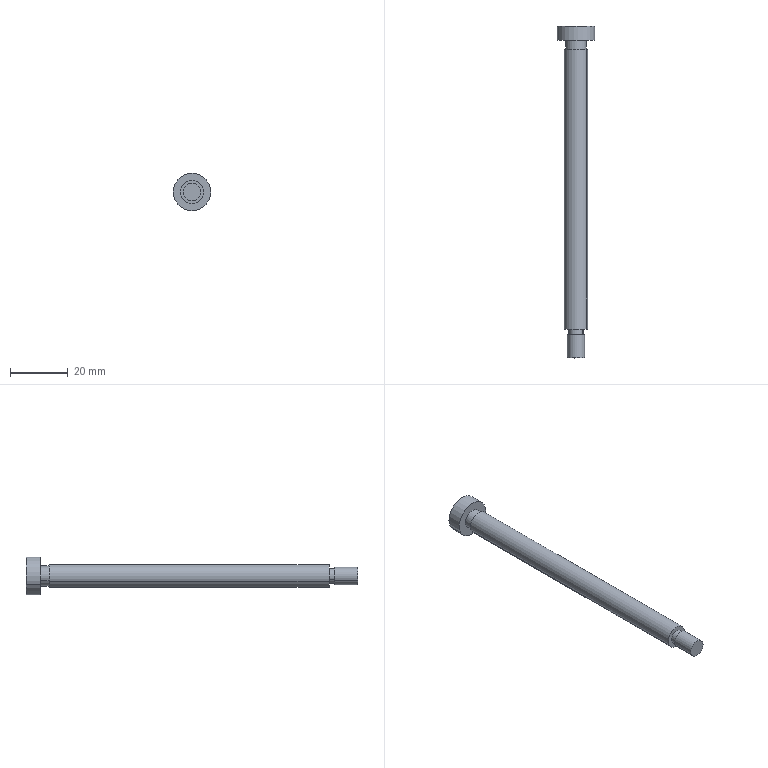Component | SolidWorks | ElectricalBoxAssembly2-1_M6-8-13-100GuidePinBolt-1 | 1 solid | 23 faces | box 13 x 115 x 13 mm | volume 5851 mm3 | plane 13 | cylinder 10 | commonest cylinder face diameters 6 x2 5 x2 13 x2 7 x2 8 x2
STEP:
#1=COLOUR_RGB('',0.7922,0.8196,0.9333);
#2=FILL_AREA_STYLE_COLOUR('',#1);
#3=FILL_AREA_STYLE('',(#2));
#4=SURFACE_STYLE_FILL_AREA(#3);
#5=SURFACE_SIDE_STYLE('',(#4));
#6=SURFACE_STYLE_USAGE(.BOTH.,#5);
#7=PRESENTATION_STYLE_ASSIGNMENT((#6));
#8=CARTESIAN_POINT('',(28.076,14.947,59.362));
#9=VERTEX_POINT('',#8);
#10=CARTESIAN_POINT('',(27.867,14.947,59.252));
#11=VERTEX_POINT('',#10);
#12=CARTESIAN_POINT('',(27.971,14.947,59.307));
#13=DIRECTION('',(0.,-1.,0.));
#14=DIRECTION('',(0.8849,0.,0.4657));
#15=AXIS2_PLACEMENT_3D('',#12,#13,#14);
#16=CIRCLE('',#15,0.1181);
#17=EDGE_CURVE('',#9,#11,#16,.T.);
#18=ORIENTED_EDGE('',*,*,#17,.F.);
#19=CARTESIAN_POINT('',(28.076,15.262,59.362));
#20=VERTEX_POINT('',#19);
#21=CARTESIAN_POINT('',(28.076,14.947,59.362));
#22=DIRECTION('',(-0.,1.,-0.));
#23=VECTOR('',#22,39.37);
#24=LINE('',#21,#23);
#25=EDGE_CURVE('',#9,#20,#24,.T.);
#26=ORIENTED_EDGE('',*,*,#25,.T.);
#27=CARTESIAN_POINT('',(27.867,15.262,59.252));
#28=VERTEX_POINT('',#27);
#29=CARTESIAN_POINT('',(27.971,15.262,59.307));
#30=DIRECTION('',(0.,-1.,0.));
#31=DIRECTION('',(0.8849,0.,0.4657));
#32=AXIS2_PLACEMENT_3D('',#29,#30,#31);
#33=CIRCLE('',#32,0.1181);
#34=EDGE_CURVE('',#20,#28,#33,.T.);
#35=ORIENTED_EDGE('',*,*,#34,.T.);
#36=CARTESIAN_POINT('',(27.867,14.947,59.252));
#37=DIRECTION('',(-0.,1.,-0.));
#38=VECTOR('',#37,39.37);
#39=LINE('',#36,#38);
#40=EDGE_CURVE('',#11,#28,#39,.T.);
#41=ORIENTED_EDGE('',*,*,#40,.F.);
#42=EDGE_LOOP('',(#18,#26,#35,#41));
#43=FACE_OUTER_BOUND('',#42,.T.);
#44=CARTESIAN_POINT('',(27.971,14.947,59.307));
#45=DIRECTION('',(-0.,1.,-0.));
#46=DIRECTION('',(-0.8849,0.,-0.4657));
#47=AXIS2_PLACEMENT_3D('',#44,#45,#46);
#48=CYLINDRICAL_SURFACE('',#47,0.1181);
#49=ADVANCED_FACE('',(#43),#48,.T.);
#50=CARTESIAN_POINT('',(28.058,15.262,59.353));
#51=VERTEX_POINT('',#50);
#52=CARTESIAN_POINT('',(27.884,15.262,59.261));
#53=VERTEX_POINT('',#52);
#54=CARTESIAN_POINT('',(27.971,15.262,59.307));
#55=DIRECTION('',(0.,-1.,0.));
#56=DIRECTION('',(0.8849,0.,0.4657));
#57=AXIS2_PLACEMENT_3D('',#54,#55,#56);
#58=CIRCLE('',#57,0.09843);
#59=EDGE_CURVE('',#51,#53,#58,.T.);
#60=ORIENTED_EDGE('',*,*,#59,.F.);
#61=CARTESIAN_POINT('',(28.058,15.341,59.353));
#62=VERTEX_POINT('',#61);
#63=CARTESIAN_POINT('',(28.058,15.262,59.353));
#64=DIRECTION('',(-0.,1.,-0.));
#65=VECTOR('',#64,39.37);
#66=LINE('',#63,#65);
#67=EDGE_CURVE('',#51,#62,#66,.T.);
#68=ORIENTED_EDGE('',*,*,#67,.T.);
#69=CARTESIAN_POINT('',(27.884,15.341,59.261));
#70=VERTEX_POINT('',#69);
#71=CARTESIAN_POINT('',(27.971,15.341,59.307));
#72=DIRECTION('',(0.,-1.,0.));
#73=DIRECTION('',(0.8849,0.,0.4657));
#74=AXIS2_PLACEMENT_3D('',#71,#72,#73);
#75=CIRCLE('',#74,0.09843);
#76=EDGE_CURVE('',#62,#70,#75,.T.);
#77=ORIENTED_EDGE('',*,*,#76,.T.);
#78=CARTESIAN_POINT('',(27.884,15.262,59.261));
#79=DIRECTION('',(-0.,1.,-0.));
#80=VECTOR('',#79,39.37);
#81=LINE('',#78,#80);
#82=EDGE_CURVE('',#53,#70,#81,.T.);
#83=ORIENTED_EDGE('',*,*,#82,.F.);
#84=EDGE_LOOP('',(#60,#68,#77,#83));
#85=FACE_OUTER_BOUND('',#84,.T.);
#86=CARTESIAN_POINT('',(27.971,15.262,59.307));
#87=DIRECTION('',(-0.,1.,-0.));
#88=DIRECTION('',(-0.8849,0.,-0.4657));
#89=AXIS2_PLACEMENT_3D('',#86,#87,#88);
#90=CYLINDRICAL_SURFACE('',#89,0.09843);
#91=ADVANCED_FACE('',(#85),#90,.T.);
#92=CARTESIAN_POINT('',(27.745,19.278,59.188));
#93=VERTEX_POINT('',#92);
#94=CARTESIAN_POINT('',(28.198,19.278,59.426));
#95=VERTEX_POINT('',#94);
#96=CARTESIAN_POINT('',(27.971,19.278,59.307));
#97=DIRECTION('',(-0.,1.,-0.));
#98=DIRECTION('',(-0.8849,0.,-0.4657));
#99=AXIS2_PLACEMENT_3D('',#96,#97,#98);
#100=CIRCLE('',#99,0.2559);
#101=EDGE_CURVE('',#93,#95,#100,.T.);
#102=ORIENTED_EDGE('',*,*,#101,.T.);
#103=CARTESIAN_POINT('',(28.198,19.475,59.426));
#104=VERTEX_POINT('',#103);
#105=CARTESIAN_POINT('',(28.198,19.278,59.426));
#106=DIRECTION('',(-0.,1.,-0.));
#107=VECTOR('',#106,39.37);
#108=LINE('',#105,#107);
#109=EDGE_CURVE('',#95,#104,#108,.T.);
#110=ORIENTED_EDGE('',*,*,#109,.T.);
#111=CARTESIAN_POINT('',(27.745,19.475,59.188));
#112=VERTEX_POINT('',#111);
#113=CARTESIAN_POINT('',(27.971,19.475,59.307));
#114=DIRECTION('',(-0.,1.,-0.));
#115=DIRECTION('',(-0.8849,0.,-0.4657));
#116=AXIS2_PLACEMENT_3D('',#113,#114,#115);
#117=CIRCLE('',#116,0.2559);
#118=EDGE_CURVE('',#112,#104,#117,.T.);
#119=ORIENTED_EDGE('',*,*,#118,.F.);
#120=CARTESIAN_POINT('',(27.745,19.278,59.188));
#121=DIRECTION('',(-0.,1.,-0.));
#122=VECTOR('',#121,39.37);
#123=LINE('',#120,#122);
#124=EDGE_CURVE('',#93,#112,#123,.T.);
#125=ORIENTED_EDGE('',*,*,#124,.F.);
#126=EDGE_LOOP('',(#102,#110,#119,#125));
#127=FACE_OUTER_BOUND('',#126,.T.);
#128=CARTESIAN_POINT('',(27.971,19.278,59.307));
#129=DIRECTION('',(-0.,1.,-0.));
#130=DIRECTION('',(-0.8849,0.,-0.4657));
#131=AXIS2_PLACEMENT_3D('',#128,#129,#130);
#132=CYLINDRICAL_SURFACE('',#131,0.2559);
#133=ADVANCED_FACE('',(#127),#132,.T.);
#134=CARTESIAN_POINT('',(28.093,19.16,59.371));
#135=VERTEX_POINT('',#134);
#136=CARTESIAN_POINT('',(27.849,19.16,59.243));
#137=VERTEX_POINT('',#136);
#138=CARTESIAN_POINT('',(27.971,19.16,59.307));
#139=DIRECTION('',(0.,-1.,0.));
#140=DIRECTION('',(0.8849,0.,0.4657));
#141=AXIS2_PLACEMENT_3D('',#138,#139,#140);
#142=CIRCLE('',#141,0.1378);
#143=EDGE_CURVE('',#135,#137,#142,.T.);
#144=ORIENTED_EDGE('',*,*,#143,.F.);
#145=CARTESIAN_POINT('',(28.093,19.278,59.371));
#146=VERTEX_POINT('',#145);
#147=CARTESIAN_POINT('',(28.093,19.16,59.371));
#148=DIRECTION('',(-0.,1.,-0.));
#149=VECTOR('',#148,39.37);
#150=LINE('',#147,#149);
#151=EDGE_CURVE('',#135,#146,#150,.T.);
#152=ORIENTED_EDGE('',*,*,#151,.T.);
#153=CARTESIAN_POINT('',(27.849,19.278,59.243));
#154=VERTEX_POINT('',#153);
#155=CARTESIAN_POINT('',(27.971,19.278,59.307));
#156=DIRECTION('',(0.,-1.,0.));
#157=DIRECTION('',(0.8849,0.,0.4657));
#158=AXIS2_PLACEMENT_3D('',#155,#156,#157);
#159=CIRCLE('',#158,0.1378);
#160=EDGE_CURVE('',#146,#154,#159,.T.);
#161=ORIENTED_EDGE('',*,*,#160,.T.);
#162=CARTESIAN_POINT('',(27.849,19.16,59.243));
#163=DIRECTION('',(-0.,1.,-0.));
#164=VECTOR('',#163,39.37);
#165=LINE('',#162,#164);
#166=EDGE_CURVE('',#137,#154,#165,.T.);
#167=ORIENTED_EDGE('',*,*,#166,.F.);
#168=EDGE_LOOP('',(#144,#152,#161,#167));
#169=FACE_OUTER_BOUND('',#168,.T.);
#170=CARTESIAN_POINT('',(27.971,19.16,59.307));
#171=DIRECTION('',(-0.,1.,-0.));
#172=DIRECTION('',(-0.8849,0.,-0.4657));
#173=AXIS2_PLACEMENT_3D('',#170,#171,#172);
#174=CYLINDRICAL_SURFACE('',#173,0.1378);
#175=ADVANCED_FACE('',(#169),#174,.T.);
#176=CARTESIAN_POINT('',(28.111,15.341,59.38));
#177=VERTEX_POINT('',#176);
#178=CARTESIAN_POINT('',(27.832,15.341,59.234));
#179=VERTEX_POINT('',#178);
#180=CARTESIAN_POINT('',(27.971,15.341,59.307));
#181=DIRECTION('',(0.,-1.,0.));
#182=DIRECTION('',(0.8849,0.,0.4657));
#183=AXIS2_PLACEMENT_3D('',#180,#181,#182);
#184=CIRCLE('',#183,0.1575);
#185=EDGE_CURVE('',#177,#179,#184,.T.);
#186=ORIENTED_EDGE('',*,*,#185,.F.);
#187=CARTESIAN_POINT('',(28.111,19.16,59.38));
#188=VERTEX_POINT('',#187);
#189=CARTESIAN_POINT('',(28.111,15.341,59.38));
#190=DIRECTION('',(-0.,1.,-0.));
#191=VECTOR('',#190,39.37);
#192=LINE('',#189,#191);
#193=EDGE_CURVE('',#177,#188,#192,.T.);
#194=ORIENTED_EDGE('',*,*,#193,.T.);
#195=CARTESIAN_POINT('',(27.832,19.16,59.234));
#196=VERTEX_POINT('',#195);
#197=CARTESIAN_POINT('',(27.971,19.16,59.307));
#198=DIRECTION('',(0.,-1.,0.));
#199=DIRECTION('',(0.8849,0.,0.4657));
#200=AXIS2_PLACEMENT_3D('',#197,#198,#199);
#201=CIRCLE('',#200,0.1575);
#202=EDGE_CURVE('',#188,#196,#201,.T.);
#203=ORIENTED_EDGE('',*,*,#202,.T.);
#204=CARTESIAN_POINT('',(27.832,15.341,59.234));
#205=DIRECTION('',(-0.,1.,-0.));
#206=VECTOR('',#205,39.37);
#207=LINE('',#204,#206);
#208=EDGE_CURVE('',#179,#196,#207,.T.);
#209=ORIENTED_EDGE('',*,*,#208,.F.);
#210=EDGE_LOOP('',(#186,#194,#203,#209));
#211=FACE_OUTER_BOUND('',#210,.T.);
#212=CARTESIAN_POINT('',(27.971,15.341,59.307));
#213=DIRECTION('',(-0.,1.,-0.));
#214=DIRECTION('',(-0.8849,0.,-0.4657));
#215=AXIS2_PLACEMENT_3D('',#212,#213,#214);
#216=CYLINDRICAL_SURFACE('',#215,0.1575);
#217=ADVANCED_FACE('',(#211),#216,.T.);
#218=CARTESIAN_POINT('',(27.971,15.341,59.307));
#219=DIRECTION('',(0.,-1.,0.));
#220=DIRECTION('',(0.8849,0.,0.4657));
#221=AXIS2_PLACEMENT_3D('',#218,#219,#220);
#222=CIRCLE('',#221,0.1575);
#223=EDGE_CURVE('',#179,#177,#222,.T.);
#224=ORIENTED_EDGE('',*,*,#223,.T.);
#225=ORIENTED_EDGE('',*,*,#185,.T.);
#226=EDGE_LOOP('',(#224,#225));
#227=FACE_OUTER_BOUND('',#226,.T.);
#228=CARTESIAN_POINT('',(27.971,15.341,59.307));
#229=DIRECTION('',(0.,-1.,0.));
#230=DIRECTION('',(0.8849,0.,0.4657));
#231=AXIS2_PLACEMENT_3D('',#228,#229,#230);
#232=CIRCLE('',#231,0.09843);
#233=EDGE_CURVE('',#70,#62,#232,.T.);
#234=ORIENTED_EDGE('',*,*,#233,.F.);
#235=ORIENTED_EDGE('',*,*,#76,.F.);
#236=EDGE_LOOP('',(#234,#235));
#237=FACE_BOUND('',#236,.T.);
#238=CARTESIAN_POINT('',(27.971,15.341,59.307));
#239=DIRECTION('',(0.,-1.,0.));
#240=DIRECTION('',(0.8849,0.,0.4657));
#241=AXIS2_PLACEMENT_3D('',#238,#239,#240);
#242=PLANE('',#241);
#243=ADVANCED_FACE('',(#227,#237),#242,.T.);
#244=ORIENTED_EDGE('',*,*,#193,.F.);
#245=ORIENTED_EDGE('',*,*,#223,.F.);
#246=ORIENTED_EDGE('',*,*,#208,.T.);
#247=CARTESIAN_POINT('',(27.971,19.16,59.307));
#248=DIRECTION('',(0.,-1.,0.));
#249=DIRECTION('',(0.8849,0.,0.4657));
#250=AXIS2_PLACEMENT_3D('',#247,#248,#249);
#251=CIRCLE('',#250,0.1575);
#252=EDGE_CURVE('',#196,#188,#251,.T.);
#253=ORIENTED_EDGE('',*,*,#252,.T.);
#254=EDGE_LOOP('',(#244,#245,#246,#253));
#255=FACE_OUTER_BOUND('',#254,.T.);
#256=CARTESIAN_POINT('',(27.971,15.341,59.307));
#257=DIRECTION('',(-0.,1.,-0.));
#258=DIRECTION('',(-0.8849,0.,-0.4657));
#259=AXIS2_PLACEMENT_3D('',#256,#257,#258);
#260=CYLINDRICAL_SURFACE('',#259,0.1575);
#261=ADVANCED_FACE('',(#255),#260,.T.);
#262=ORIENTED_EDGE('',*,*,#252,.F.);
#263=ORIENTED_EDGE('',*,*,#202,.F.);
#264=EDGE_LOOP('',(#262,#263));
#265=FACE_OUTER_BOUND('',#264,.T.);
#266=CARTESIAN_POINT('',(27.971,19.16,59.307));
#267=DIRECTION('',(0.,-1.,0.));
#268=DIRECTION('',(0.8849,0.,0.4657));
#269=AXIS2_PLACEMENT_3D('',#266,#267,#268);
#270=CIRCLE('',#269,0.1378);
#271=EDGE_CURVE('',#137,#135,#270,.T.);
#272=ORIENTED_EDGE('',*,*,#271,.T.);
#273=ORIENTED_EDGE('',*,*,#143,.T.);
#274=EDGE_LOOP('',(#272,#273));
#275=FACE_BOUND('',#274,.T.);
#276=CARTESIAN_POINT('',(27.971,19.16,59.307));
#277=DIRECTION('',(0.,-1.,0.));
#278=DIRECTION('',(0.8849,0.,0.4657));
#279=AXIS2_PLACEMENT_3D('',#276,#277,#278);
#280=PLANE('',#279);
#281=ADVANCED_FACE('',(#265,#275),#280,.F.);
#282=ORIENTED_EDGE('',*,*,#151,.F.);
#283=ORIENTED_EDGE('',*,*,#271,.F.);
#284=ORIENTED_EDGE('',*,*,#166,.T.);
#285=CARTESIAN_POINT('',(27.971,19.278,59.307));
#286=DIRECTION('',(0.,-1.,0.));
#287=DIRECTION('',(0.8849,0.,0.4657));
#288=AXIS2_PLACEMENT_3D('',#285,#286,#287);
#289=CIRCLE('',#288,0.1378);
#290=EDGE_CURVE('',#154,#146,#289,.T.);
#291=ORIENTED_EDGE('',*,*,#290,.T.);
#292=EDGE_LOOP('',(#282,#283,#284,#291));
#293=FACE_OUTER_BOUND('',#292,.T.);
#294=CARTESIAN_POINT('',(27.971,19.16,59.307));
#295=DIRECTION('',(-0.,1.,-0.));
#296=DIRECTION('',(-0.8849,0.,-0.4657));
#297=AXIS2_PLACEMENT_3D('',#294,#295,#296);
#298=CYLINDRICAL_SURFACE('',#297,0.1378);
#299=ADVANCED_FACE('',(#293),#298,.T.);
#300=CARTESIAN_POINT('',(27.968,19.475,59.216));
#301=VERTEX_POINT('',#300);
#302=CARTESIAN_POINT('',(27.891,19.475,59.265));
#303=VERTEX_POINT('',#302);
#304=CARTESIAN_POINT('',(27.968,19.475,59.216));
#305=DIRECTION('',(-0.8458,0.,0.5335));
#306=VECTOR('',#305,39.37);
#307=LINE('',#304,#306);
#308=EDGE_CURVE('',#301,#303,#307,.T.);
#309=ORIENTED_EDGE('',*,*,#308,.F.);
#310=CARTESIAN_POINT('',(28.048,19.475,59.259));
#311=VERTEX_POINT('',#310);
#312=CARTESIAN_POINT('',(28.048,19.475,59.259));
#313=DIRECTION('',(-0.8849,-0.,-0.4657));
#314=VECTOR('',#313,39.37);
#315=LINE('',#312,#314);
#316=EDGE_CURVE('',#311,#301,#315,.T.);
#317=ORIENTED_EDGE('',*,*,#316,.F.);
#318=CARTESIAN_POINT('',(28.052,19.475,59.349));
#319=VERTEX_POINT('',#318);
#320=CARTESIAN_POINT('',(28.052,19.475,59.349));
#321=DIRECTION('',(-0.03914,-0.,-0.9992));
#322=VECTOR('',#321,39.37);
#323=LINE('',#320,#322);
#324=EDGE_CURVE('',#319,#311,#323,.T.);
#325=ORIENTED_EDGE('',*,*,#324,.F.);
#326=CARTESIAN_POINT('',(27.975,19.475,59.398));
#327=VERTEX_POINT('',#326);
#328=CARTESIAN_POINT('',(27.975,19.475,59.398));
#329=DIRECTION('',(0.8458,-0.,-0.5335));
#330=VECTOR('',#329,39.37);
#331=LINE('',#328,#330);
#332=EDGE_CURVE('',#327,#319,#331,.T.);
#333=ORIENTED_EDGE('',*,*,#332,.F.);
#334=CARTESIAN_POINT('',(27.894,19.475,59.356));
#335=VERTEX_POINT('',#334);
#336=CARTESIAN_POINT('',(27.894,19.475,59.356));
#337=DIRECTION('',(0.8849,0.,0.4657));
#338=VECTOR('',#337,39.37);
#339=LINE('',#336,#338);
#340=EDGE_CURVE('',#335,#327,#339,.T.);
#341=ORIENTED_EDGE('',*,*,#340,.F.);
#342=CARTESIAN_POINT('',(27.891,19.475,59.265));
#343=DIRECTION('',(0.03914,0.,0.9992));
#344=VECTOR('',#343,39.37);
#345=LINE('',#342,#344);
#346=EDGE_CURVE('',#303,#335,#345,.T.);
#347=ORIENTED_EDGE('',*,*,#346,.F.);
#348=EDGE_LOOP('',(#309,#317,#325,#333,#341,#347));
#349=FACE_BOUND('',#348,.T.);
#350=ORIENTED_EDGE('',*,*,#118,.T.);
#351=CARTESIAN_POINT('',(27.971,19.475,59.307));
#352=DIRECTION('',(-0.,1.,-0.));
#353=DIRECTION('',(-0.8849,0.,-0.4657));
#354=AXIS2_PLACEMENT_3D('',#351,#352,#353);
#355=CIRCLE('',#354,0.2559);
#356=EDGE_CURVE('',#104,#112,#355,.T.);
#357=ORIENTED_EDGE('',*,*,#356,.T.);
#358=EDGE_LOOP('',(#350,#357));
#359=FACE_OUTER_BOUND('',#358,.T.);
#360=CARTESIAN_POINT('',(27.971,19.475,59.307));
#361=DIRECTION('',(-0.,1.,-0.));
#362=DIRECTION('',(-0.8849,-0.,-0.4657));
#363=AXIS2_PLACEMENT_3D('',#360,#361,#362);
#364=PLANE('',#363);
#365=ADVANCED_FACE('',(#349,#359),#364,.T.);
#366=ORIENTED_EDGE('',*,*,#109,.F.);
#367=CARTESIAN_POINT('',(27.971,19.278,59.307));
#368=DIRECTION('',(-0.,1.,-0.));
#369=DIRECTION('',(-0.8849,0.,-0.4657));
#370=AXIS2_PLACEMENT_3D('',#367,#368,#369);
#371=CIRCLE('',#370,0.2559);
#372=EDGE_CURVE('',#95,#93,#371,.T.);
#373=ORIENTED_EDGE('',*,*,#372,.T.);
#374=ORIENTED_EDGE('',*,*,#124,.T.);
#375=ORIENTED_EDGE('',*,*,#356,.F.);
#376=EDGE_LOOP('',(#366,#373,#374,#375));
#377=FACE_OUTER_BOUND('',#376,.T.);
#378=CARTESIAN_POINT('',(27.971,19.278,59.307));
#379=DIRECTION('',(-0.,1.,-0.));
#380=DIRECTION('',(-0.8849,0.,-0.4657));
#381=AXIS2_PLACEMENT_3D('',#378,#379,#380);
#382=CYLINDRICAL_SURFACE('',#381,0.2559);
#383=ADVANCED_FACE('',(#377),#382,.T.);
#384=ORIENTED_EDGE('',*,*,#101,.F.);
#385=ORIENTED_EDGE('',*,*,#372,.F.);
#386=EDGE_LOOP('',(#384,#385));
#387=FACE_OUTER_BOUND('',#386,.T.);
#388=ORIENTED_EDGE('',*,*,#290,.F.);
#389=ORIENTED_EDGE('',*,*,#160,.F.);
#390=EDGE_LOOP('',(#388,#389));
#391=FACE_BOUND('',#390,.T.);
#392=CARTESIAN_POINT('',(27.971,19.278,59.307));
#393=DIRECTION('',(-0.,1.,-0.));
#394=DIRECTION('',(-0.8849,-0.,-0.4657));
#395=AXIS2_PLACEMENT_3D('',#392,#393,#394);
#396=PLANE('',#395);
#397=ADVANCED_FACE('',(#387,#391),#396,.F.);
#398=CARTESIAN_POINT('',(27.971,15.262,59.307));
#399=DIRECTION('',(0.,-1.,0.));
#400=DIRECTION('',(0.8849,0.,0.4657));
#401=AXIS2_PLACEMENT_3D('',#398,#399,#400);
#402=CIRCLE('',#401,0.1181);
#403=EDGE_CURVE('',#28,#20,#402,.T.);
#404=ORIENTED_EDGE('',*,*,#403,.F.);
#405=ORIENTED_EDGE('',*,*,#34,.F.);
#406=EDGE_LOOP('',(#404,#405));
#407=FACE_OUTER_BOUND('',#406,.T.);
#408=CARTESIAN_POINT('',(27.971,15.262,59.307));
#409=DIRECTION('',(0.,-1.,0.));
#410=DIRECTION('',(0.8849,0.,0.4657));
#411=AXIS2_PLACEMENT_3D('',#408,#409,#410);
#412=CIRCLE('',#411,0.09843);
#413=EDGE_CURVE('',#53,#51,#412,.T.);
#414=ORIENTED_EDGE('',*,*,#413,.T.);
#415=ORIENTED_EDGE('',*,*,#59,.T.);
#416=EDGE_LOOP('',(#414,#415));
#417=FACE_BOUND('',#416,.T.);
#418=CARTESIAN_POINT('',(27.971,15.262,59.307));
#419=DIRECTION('',(0.,-1.,0.));
#420=DIRECTION('',(0.8849,0.,0.4657));
#421=AXIS2_PLACEMENT_3D('',#418,#419,#420);
#422=PLANE('',#421);
#423=ADVANCED_FACE('',(#407,#417),#422,.F.);
#424=ORIENTED_EDGE('',*,*,#67,.F.);
#425=ORIENTED_EDGE('',*,*,#413,.F.);
#426=ORIENTED_EDGE('',*,*,#82,.T.);
#427=ORIENTED_EDGE('',*,*,#233,.T.);
#428=EDGE_LOOP('',(#424,#425,#426,#427));
#429=FACE_OUTER_BOUND('',#428,.T.);
#430=CARTESIAN_POINT('',(27.971,15.262,59.307));
#431=DIRECTION('',(-0.,1.,-0.));
#432=DIRECTION('',(-0.8849,0.,-0.4657));
#433=AXIS2_PLACEMENT_3D('',#430,#431,#432);
#434=CYLINDRICAL_SURFACE('',#433,0.09843);
#435=ADVANCED_FACE('',(#429),#434,.T.);
#436=CARTESIAN_POINT('',(27.971,14.947,59.307));
#437=DIRECTION('',(0.,-1.,0.));
#438=DIRECTION('',(0.8849,0.,0.4657));
#439=AXIS2_PLACEMENT_3D('',#436,#437,#438);
#440=CIRCLE('',#439,0.1181);
#441=EDGE_CURVE('',#11,#9,#440,.T.);
#442=ORIENTED_EDGE('',*,*,#441,.T.);
#443=ORIENTED_EDGE('',*,*,#17,.T.);
#444=EDGE_LOOP('',(#442,#443));
#445=FACE_OUTER_BOUND('',#444,.T.);
#446=CARTESIAN_POINT('',(27.971,14.947,59.307));
#447=DIRECTION('',(0.,-1.,0.));
#448=DIRECTION('',(0.8849,0.,0.4657));
#449=AXIS2_PLACEMENT_3D('',#446,#447,#448);
#450=PLANE('',#449);
#451=ADVANCED_FACE('',(#445),#450,.T.);
#452=ORIENTED_EDGE('',*,*,#25,.F.);
#453=ORIENTED_EDGE('',*,*,#441,.F.);
#454=ORIENTED_EDGE('',*,*,#40,.T.);
#455=ORIENTED_EDGE('',*,*,#403,.T.);
#456=EDGE_LOOP('',(#452,#453,#454,#455));
#457=FACE_OUTER_BOUND('',#456,.T.);
#458=CARTESIAN_POINT('',(27.971,14.947,59.307));
#459=DIRECTION('',(-0.,1.,-0.));
#460=DIRECTION('',(-0.8849,0.,-0.4657));
#461=AXIS2_PLACEMENT_3D('',#458,#459,#460);
#462=CYLINDRICAL_SURFACE('',#461,0.1181);
#463=ADVANCED_FACE('',(#457),#462,.T.);
#464=ORIENTED_EDGE('',*,*,#308,.T.);
#465=CARTESIAN_POINT('',(27.891,19.278,59.265));
#466=VERTEX_POINT('',#465);
#467=CARTESIAN_POINT('',(27.891,19.278,59.265));
#468=DIRECTION('',(-0.,1.,-0.));
#469=VECTOR('',#468,39.37);
#470=LINE('',#467,#469);
#471=EDGE_CURVE('',#466,#303,#470,.T.);
#472=ORIENTED_EDGE('',*,*,#471,.F.);
#473=CARTESIAN_POINT('',(27.968,19.278,59.216));
#474=VERTEX_POINT('',#473);
#475=CARTESIAN_POINT('',(27.968,19.278,59.216));
#476=DIRECTION('',(-0.8458,0.,0.5335));
#477=VECTOR('',#476,39.37);
#478=LINE('',#475,#477);
#479=EDGE_CURVE('',#474,#466,#478,.T.);
#480=ORIENTED_EDGE('',*,*,#479,.F.);
#481=CARTESIAN_POINT('',(27.968,19.278,59.216));
#482=DIRECTION('',(-0.,1.,-0.));
#483=VECTOR('',#482,39.37);
#484=LINE('',#481,#483);
#485=EDGE_CURVE('',#474,#301,#484,.T.);
#486=ORIENTED_EDGE('',*,*,#485,.T.);
#487=EDGE_LOOP('',(#464,#472,#480,#486));
#488=FACE_OUTER_BOUND('',#487,.T.);
#489=CARTESIAN_POINT('',(27.968,19.278,59.216));
#490=DIRECTION('',(-0.5335,-0.,-0.8458));
#491=DIRECTION('',(-0.8458,0.,0.5335));
#492=AXIS2_PLACEMENT_3D('',#489,#490,#491);
#493=PLANE('',#492);
#494=ADVANCED_FACE('',(#488),#493,.F.);
#495=ORIENTED_EDGE('',*,*,#316,.T.);
#496=ORIENTED_EDGE('',*,*,#485,.F.);
#497=CARTESIAN_POINT('',(28.048,19.278,59.259));
#498=VERTEX_POINT('',#497);
#499=CARTESIAN_POINT('',(28.048,19.278,59.259));
#500=DIRECTION('',(-0.8849,-0.,-0.4657));
#501=VECTOR('',#500,39.37);
#502=LINE('',#499,#501);
#503=EDGE_CURVE('',#498,#474,#502,.T.);
#504=ORIENTED_EDGE('',*,*,#503,.F.);
#505=CARTESIAN_POINT('',(28.048,19.278,59.259));
#506=DIRECTION('',(-0.,1.,-0.));
#507=VECTOR('',#506,39.37);
#508=LINE('',#505,#507);
#509=EDGE_CURVE('',#498,#311,#508,.T.);
#510=ORIENTED_EDGE('',*,*,#509,.T.);
#511=EDGE_LOOP('',(#495,#496,#504,#510));
#512=FACE_OUTER_BOUND('',#511,.T.);
#513=CARTESIAN_POINT('',(28.048,19.278,59.259));
#514=DIRECTION('',(0.4657,-0.,-0.8849));
#515=DIRECTION('',(-0.8849,-0.,-0.4657));
#516=AXIS2_PLACEMENT_3D('',#513,#514,#515);
#517=PLANE('',#516);
#518=ADVANCED_FACE('',(#512),#517,.F.);
#519=ORIENTED_EDGE('',*,*,#324,.T.);
#520=ORIENTED_EDGE('',*,*,#509,.F.);
#521=CARTESIAN_POINT('',(28.052,19.278,59.349));
#522=VERTEX_POINT('',#521);
#523=CARTESIAN_POINT('',(28.052,19.278,59.349));
#524=DIRECTION('',(-0.03914,-0.,-0.9992));
#525=VECTOR('',#524,39.37);
#526=LINE('',#523,#525);
#527=EDGE_CURVE('',#522,#498,#526,.T.);
#528=ORIENTED_EDGE('',*,*,#527,.F.);
#529=CARTESIAN_POINT('',(28.052,19.278,59.349));
#530=DIRECTION('',(-0.,1.,-0.));
#531=VECTOR('',#530,39.37);
#532=LINE('',#529,#531);
#533=EDGE_CURVE('',#522,#319,#532,.T.);
#534=ORIENTED_EDGE('',*,*,#533,.T.);
#535=EDGE_LOOP('',(#519,#520,#528,#534));
#536=FACE_OUTER_BOUND('',#535,.T.);
#537=CARTESIAN_POINT('',(28.052,19.278,59.349));
#538=DIRECTION('',(0.9992,0.,-0.03914));
#539=DIRECTION('',(-0.03914,-0.,-0.9992));
#540=AXIS2_PLACEMENT_3D('',#537,#538,#539);
#541=PLANE('',#540);
#542=ADVANCED_FACE('',(#536),#541,.F.);
#543=ORIENTED_EDGE('',*,*,#332,.T.);
#544=ORIENTED_EDGE('',*,*,#533,.F.);
#545=CARTESIAN_POINT('',(27.975,19.278,59.398));
#546=VERTEX_POINT('',#545);
#547=CARTESIAN_POINT('',(27.975,19.278,59.398));
#548=DIRECTION('',(0.8458,-0.,-0.5335));
#549=VECTOR('',#548,39.37);
#550=LINE('',#547,#549);
#551=EDGE_CURVE('',#546,#522,#550,.T.);
#552=ORIENTED_EDGE('',*,*,#551,.F.);
#553=CARTESIAN_POINT('',(27.975,19.278,59.398));
#554=DIRECTION('',(-0.,1.,-0.));
#555=VECTOR('',#554,39.37);
#556=LINE('',#553,#555);
#557=EDGE_CURVE('',#546,#327,#556,.T.);
#558=ORIENTED_EDGE('',*,*,#557,.T.);
#559=EDGE_LOOP('',(#543,#544,#552,#558));
#560=FACE_OUTER_BOUND('',#559,.T.);
#561=CARTESIAN_POINT('',(27.975,19.278,59.398));
#562=DIRECTION('',(0.5335,0.,0.8458));
#563=DIRECTION('',(0.8458,-0.,-0.5335));
#564=AXIS2_PLACEMENT_3D('',#561,#562,#563);
#565=PLANE('',#564);
#566=ADVANCED_FACE('',(#560),#565,.F.);
#567=ORIENTED_EDGE('',*,*,#340,.T.);
#568=ORIENTED_EDGE('',*,*,#557,.F.);
#569=CARTESIAN_POINT('',(27.894,19.278,59.356));
#570=VERTEX_POINT('',#569);
#571=CARTESIAN_POINT('',(27.894,19.278,59.356));
#572=DIRECTION('',(0.8849,0.,0.4657));
#573=VECTOR('',#572,39.37);
#574=LINE('',#571,#573);
#575=EDGE_CURVE('',#570,#546,#574,.T.);
#576=ORIENTED_EDGE('',*,*,#575,.F.);
#577=CARTESIAN_POINT('',(27.894,19.278,59.356));
#578=DIRECTION('',(-0.,1.,-0.));
#579=VECTOR('',#578,39.37);
#580=LINE('',#577,#579);
#581=EDGE_CURVE('',#570,#335,#580,.T.);
#582=ORIENTED_EDGE('',*,*,#581,.T.);
#583=EDGE_LOOP('',(#567,#568,#576,#582));
#584=FACE_OUTER_BOUND('',#583,.T.);
#585=CARTESIAN_POINT('',(27.894,19.278,59.356));
#586=DIRECTION('',(-0.4657,0.,0.8849));
#587=DIRECTION('',(-0.,1.,-0.));
#588=AXIS2_PLACEMENT_3D('',#585,#586,#587);
#589=PLANE('',#588);
#590=ADVANCED_FACE('',(#584),#589,.F.);
#591=ORIENTED_EDGE('',*,*,#346,.T.);
#592=ORIENTED_EDGE('',*,*,#581,.F.);
#593=CARTESIAN_POINT('',(27.891,19.278,59.265));
#594=DIRECTION('',(0.03914,0.,0.9992));
#595=VECTOR('',#594,39.37);
#596=LINE('',#593,#595);
#597=EDGE_CURVE('',#466,#570,#596,.T.);
#598=ORIENTED_EDGE('',*,*,#597,.F.);
#599=ORIENTED_EDGE('',*,*,#471,.T.);
#600=EDGE_LOOP('',(#591,#592,#598,#599));
#601=FACE_OUTER_BOUND('',#600,.T.);
#602=CARTESIAN_POINT('',(27.891,19.278,59.265));
#603=DIRECTION('',(-0.9992,-0.,0.03914));
#604=DIRECTION('',(0.03914,0.,0.9992));
#605=AXIS2_PLACEMENT_3D('',#602,#603,#604);
#606=PLANE('',#605);
#607=ADVANCED_FACE('',(#601),#606,.F.);
#608=ORIENTED_EDGE('',*,*,#479,.T.);
#609=ORIENTED_EDGE('',*,*,#597,.T.);
#610=ORIENTED_EDGE('',*,*,#575,.T.);
#611=ORIENTED_EDGE('',*,*,#551,.T.);
#612=ORIENTED_EDGE('',*,*,#527,.T.);
#613=ORIENTED_EDGE('',*,*,#503,.T.);
#614=EDGE_LOOP('',(#608,#609,#610,#611,#612,#613));
#615=FACE_OUTER_BOUND('',#614,.T.);
#616=CARTESIAN_POINT('',(27.971,19.278,59.307));
#617=DIRECTION('',(-0.,1.,-0.));
#618=DIRECTION('',(-0.8849,-0.,-0.4657));
#619=AXIS2_PLACEMENT_3D('',#616,#617,#618);
#620=PLANE('',#619);
#621=ADVANCED_FACE('',(#615),#620,.T.);
#622=CLOSED_SHELL('',(#49,#91,#133,#175,#217,#243,#261,#281,#299,#365,#383,#397,#423,#435,#451,#463,#494,#518,#542,#566,#590,#607,#621));
#623=MANIFOLD_SOLID_BREP('',#622);
#624=STYLED_ITEM('',(#7),#623);
#625=PRESENTATION_LAYER_ASSIGNMENT('','',(#624));
#626=CARTESIAN_POINT('',(0.,0.,0.));
#627=DIRECTION('',(0.,0.,1.));
#628=DIRECTION('',(1.,0.,0.));
#629=AXIS2_PLACEMENT_3D('',#626,#627,#628);
#630=(LENGTH_UNIT()NAMED_UNIT(*)SI_UNIT($,.METRE.));
#631=LENGTH_MEASURE_WITH_UNIT(LENGTH_MEASURE(0.0254),#630);
#632=DIMENSIONAL_EXPONENTS(1.,0.,0.,0.,0.,0.,0.);
#633=(CONVERSION_BASED_UNIT('',#631)LENGTH_UNIT()NAMED_UNIT(#632));
#634=UNCERTAINTY_MEASURE_WITH_UNIT(LENGTH_MEASURE(0.00001),#633,'','');
#635=(NAMED_UNIT(*)PLANE_ANGLE_UNIT()SI_UNIT($,.RADIAN.));
#636=(NAMED_UNIT(*)SI_UNIT($,.STERADIAN.)SOLID_ANGLE_UNIT());
#637=(GEOMETRIC_REPRESENTATION_CONTEXT(3)GLOBAL_UNCERTAINTY_ASSIGNED_CONTEXT((#634))GLOBAL_UNIT_ASSIGNED_CONTEXT((#633,#635,#636))REPRESENTATION_CONTEXT('',''));
#638=ADVANCED_BREP_SHAPE_REPRESENTATION('',(#623,#629),#637);
#639=(LENGTH_UNIT()NAMED_UNIT(*)SI_UNIT($,.METRE.));
#640=LENGTH_MEASURE_WITH_UNIT(LENGTH_MEASURE(0.0254),#639);
#641=DIMENSIONAL_EXPONENTS(1.,0.,0.,0.,0.,0.,0.);
#642=(CONVERSION_BASED_UNIT('',#640)LENGTH_UNIT()NAMED_UNIT(#641));
#643=UNCERTAINTY_MEASURE_WITH_UNIT(LENGTH_MEASURE(0.00001),#642,'','');
#644=(NAMED_UNIT(*)PLANE_ANGLE_UNIT()SI_UNIT($,.RADIAN.));
#645=(NAMED_UNIT(*)SI_UNIT($,.STERADIAN.)SOLID_ANGLE_UNIT());
#646=(GEOMETRIC_REPRESENTATION_CONTEXT(3)GLOBAL_UNCERTAINTY_ASSIGNED_CONTEXT((#643))GLOBAL_UNIT_ASSIGNED_CONTEXT((#642,#644,#645))REPRESENTATION_CONTEXT('',''));
#647=MECHANICAL_DESIGN_GEOMETRIC_PRESENTATION_REPRESENTATION('',(#624),#646);